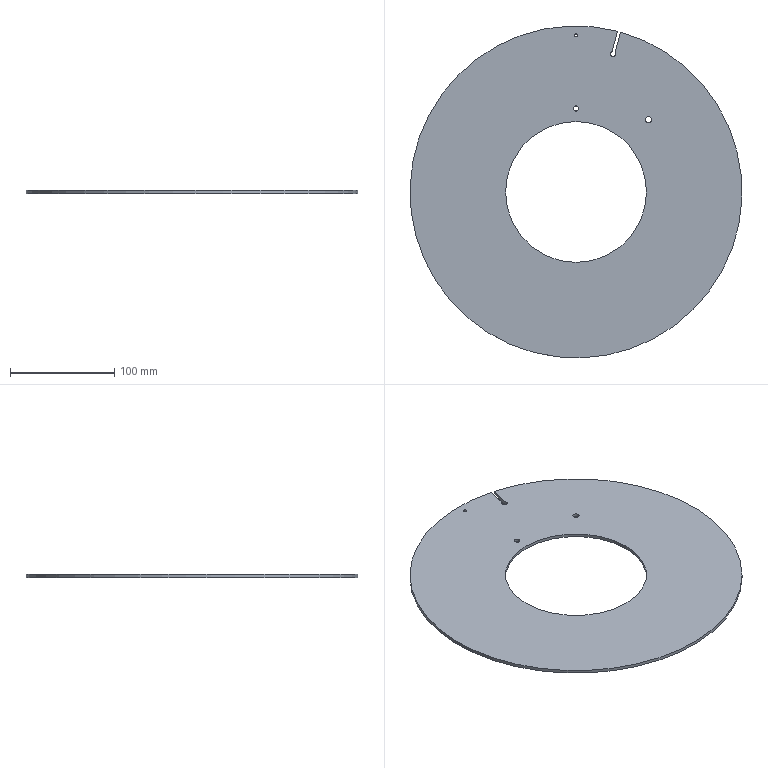Component | NX | SUPPORT_PLATE_1 | 1 solid | 10 faces | box 318 x 318 x 3 mm | volume 194925 mm3 | cylinder 6 | plane 4 | commonest cylinder face diameters 5 x2 318 x1 135 x1 6 x1 3 x1
STEP:
#1=CARTESIAN_POINT('',(0.,0.,0.));
#2=DIRECTION('',(0.,0.,1.));
#3=DIRECTION('',(1.,0.,0.));
#4=AXIS2_PLACEMENT_3D('',#1,#2,#3);
#5=CARTESIAN_POINT('',(42.599,153.187,21.));
#6=VERTEX_POINT('',#5);
#7=CARTESIAN_POINT('',(42.599,153.187,24.));
#8=VERTEX_POINT('',#7);
#9=CARTESIAN_POINT('',(42.599,153.187,20.7));
#10=DIRECTION('',(0.,0.,1.));
#11=VECTOR('',#10,1.);
#12=LINE('',#9,#11);
#13=CARTESIAN_POINT('',(0.,0.,21.));
#14=DIRECTION('',(0.,0.,1.));
#15=DIRECTION('',(1.,0.,0.));
#16=AXIS2_PLACEMENT_3D('',#13,#14,#15);
#17=CYLINDRICAL_SURFACE('',#16,159.);
#18=CARTESIAN_POINT('',(7.583,-0.3));
#19=DIRECTION('',(0.,1.));
#20=VECTOR('',#19,1.);
#21=LINE('',#18,#20);
#22=(GEOMETRIC_REPRESENTATION_CONTEXT(2)PARAMETRIC_REPRESENTATION_CONTEXT()REPRESENTATION_CONTEXT('',''));
#23=DEFINITIONAL_REPRESENTATION('',(#21),#22);
#24=PCURVE('',#17,#23);
#25=CARTESIAN_POINT('',(42.599,153.187,20.7));
#26=DIRECTION('',(-0.9659,0.2588,0.));
#27=DIRECTION('',(0.2588,0.9659,0.));
#28=AXIS2_PLACEMENT_3D('',#25,#26,#27);
#29=PLANE('',#28);
#30=CARTESIAN_POINT('',(0.,0.));
#31=DIRECTION('',(0.,-1.));
#32=VECTOR('',#31,1.);
#33=LINE('',#30,#32);
#34=(GEOMETRIC_REPRESENTATION_CONTEXT(2)PARAMETRIC_REPRESENTATION_CONTEXT()REPRESENTATION_CONTEXT('',''));
#35=DEFINITIONAL_REPRESENTATION('',(#33),#34);
#36=PCURVE('',#29,#35);
#37=SURFACE_CURVE('',#12,(#24,#36),.PCURVE_S1.);
#38=EDGE_CURVE('',#6,#8,#37,.T.);
#39=ORIENTED_EDGE('',*,*,#38,.T.);
#40=CARTESIAN_POINT('',(39.702,153.964,24.));
#41=VERTEX_POINT('',#40);
#42=CARTESIAN_POINT('',(0.,0.,24.));
#43=DIRECTION('',(0.,0.,-1.));
#44=DIRECTION('',(-1.,0.,0.));
#45=AXIS2_PLACEMENT_3D('',#42,#43,#44);
#46=CIRCLE('',#45,159.);
#47=CARTESIAN_POINT('',(9.425,3.));
#48=DIRECTION('',(-1.,0.));
#49=VECTOR('',#48,1.);
#50=LINE('',#47,#49);
#51=(GEOMETRIC_REPRESENTATION_CONTEXT(2)PARAMETRIC_REPRESENTATION_CONTEXT()REPRESENTATION_CONTEXT('',''));
#52=DEFINITIONAL_REPRESENTATION('',(#50),#51);
#53=PCURVE('',#17,#52);
#54=CARTESIAN_POINT('',(0.,0.,24.));
#55=DIRECTION('',(0.,0.,-1.));
#56=DIRECTION('',(-1.,0.,0.));
#57=AXIS2_PLACEMENT_3D('',#54,#55,#56);
#58=PLANE('',#57);
#59=CARTESIAN_POINT('',(0.,0.));
#60=DIRECTION('',(1.,0.));
#61=AXIS2_PLACEMENT_2D('',#59,#60);
#62=CIRCLE('',#61,159.);
#63=(GEOMETRIC_REPRESENTATION_CONTEXT(2)PARAMETRIC_REPRESENTATION_CONTEXT()REPRESENTATION_CONTEXT('',''));
#64=DEFINITIONAL_REPRESENTATION('',(#62),#63);
#65=PCURVE('',#58,#64);
#66=SURFACE_CURVE('',#46,(#53,#65),.PCURVE_S1.);
#67=EDGE_CURVE('',#8,#41,#66,.T.);
#68=ORIENTED_EDGE('',*,*,#67,.T.);
#69=CARTESIAN_POINT('',(39.702,153.964,21.));
#70=VERTEX_POINT('',#69);
#71=CARTESIAN_POINT('',(39.702,153.964,20.7));
#72=DIRECTION('',(0.,0.,1.));
#73=VECTOR('',#72,1.);
#74=LINE('',#71,#73);
#75=CARTESIAN_POINT('',(1.318,-0.3));
#76=DIRECTION('',(0.,1.));
#77=VECTOR('',#76,1.);
#78=LINE('',#75,#77);
#79=(GEOMETRIC_REPRESENTATION_CONTEXT(2)PARAMETRIC_REPRESENTATION_CONTEXT()REPRESENTATION_CONTEXT('',''));
#80=DEFINITIONAL_REPRESENTATION('',(#78),#79);
#81=PCURVE('',#17,#80);
#82=CARTESIAN_POINT('',(34.527,134.652,20.7));
#83=DIRECTION('',(0.9659,-0.2588,0.));
#84=DIRECTION('',(-0.2588,-0.9659,0.));
#85=AXIS2_PLACEMENT_3D('',#82,#83,#84);
#86=PLANE('',#85);
#87=CARTESIAN_POINT('',(-19.993,0.));
#88=DIRECTION('',(0.,-1.));
#89=VECTOR('',#88,1.);
#90=LINE('',#87,#89);
#91=(GEOMETRIC_REPRESENTATION_CONTEXT(2)PARAMETRIC_REPRESENTATION_CONTEXT()REPRESENTATION_CONTEXT('',''));
#92=DEFINITIONAL_REPRESENTATION('',(#90),#91);
#93=PCURVE('',#86,#92);
#94=SURFACE_CURVE('',#74,(#81,#93),.PCURVE_S1.);
#95=EDGE_CURVE('',#70,#41,#94,.T.);
#96=ORIENTED_EDGE('',*,*,#95,.F.);
#97=CARTESIAN_POINT('',(0.,0.,21.));
#98=DIRECTION('',(0.,0.,-1.));
#99=DIRECTION('',(-1.,0.,0.));
#100=AXIS2_PLACEMENT_3D('',#97,#98,#99);
#101=CIRCLE('',#100,159.);
#102=CARTESIAN_POINT('',(9.425,0.));
#103=DIRECTION('',(-1.,0.));
#104=VECTOR('',#103,1.);
#105=LINE('',#102,#104);
#106=(GEOMETRIC_REPRESENTATION_CONTEXT(2)PARAMETRIC_REPRESENTATION_CONTEXT()REPRESENTATION_CONTEXT('',''));
#107=DEFINITIONAL_REPRESENTATION('',(#105),#106);
#108=PCURVE('',#17,#107);
#109=CARTESIAN_POINT('',(0.,0.,21.));
#110=DIRECTION('',(0.,0.,-1.));
#111=DIRECTION('',(-1.,0.,0.));
#112=AXIS2_PLACEMENT_3D('',#109,#110,#111);
#113=PLANE('',#112);
#114=CARTESIAN_POINT('',(0.,0.));
#115=DIRECTION('',(1.,0.));
#116=AXIS2_PLACEMENT_2D('',#114,#115);
#117=CIRCLE('',#116,159.);
#118=(GEOMETRIC_REPRESENTATION_CONTEXT(2)PARAMETRIC_REPRESENTATION_CONTEXT()REPRESENTATION_CONTEXT('',''));
#119=DEFINITIONAL_REPRESENTATION('',(#117),#118);
#120=PCURVE('',#113,#119);
#121=SURFACE_CURVE('',#101,(#108,#120),.PCURVE_S1.);
#122=EDGE_CURVE('',#6,#70,#121,.T.);
#123=ORIENTED_EDGE('',*,*,#122,.F.);
#124=EDGE_LOOP('',(#39,#68,#96,#123));
#125=FACE_BOUND('',#124,.T.);
#126=ADVANCED_FACE('',(#125),#17,.T.);
#127=CARTESIAN_POINT('',(-67.5,0.,21.));
#128=VERTEX_POINT('',#127);
#129=CARTESIAN_POINT('',(0.,0.,21.));
#130=DIRECTION('',(0.,0.,-1.));
#131=DIRECTION('',(-1.,0.,0.));
#132=AXIS2_PLACEMENT_3D('',#129,#130,#131);
#133=CIRCLE('',#132,67.5);
#134=CARTESIAN_POINT('',(0.,0.));
#135=DIRECTION('',(1.,0.));
#136=AXIS2_PLACEMENT_2D('',#134,#135);
#137=CIRCLE('',#136,67.5);
#138=(GEOMETRIC_REPRESENTATION_CONTEXT(2)PARAMETRIC_REPRESENTATION_CONTEXT()REPRESENTATION_CONTEXT('',''));
#139=DEFINITIONAL_REPRESENTATION('',(#137),#138);
#140=PCURVE('',#113,#139);
#141=CARTESIAN_POINT('',(0.,0.,21.));
#142=DIRECTION('',(0.,0.,1.));
#143=DIRECTION('',(1.,0.,0.));
#144=AXIS2_PLACEMENT_3D('',#141,#142,#143);
#145=CYLINDRICAL_SURFACE('',#144,67.5);
#146=CARTESIAN_POINT('',(9.425,0.));
#147=DIRECTION('',(-1.,0.));
#148=VECTOR('',#147,1.);
#149=LINE('',#146,#148);
#150=(GEOMETRIC_REPRESENTATION_CONTEXT(2)PARAMETRIC_REPRESENTATION_CONTEXT()REPRESENTATION_CONTEXT('',''));
#151=DEFINITIONAL_REPRESENTATION('',(#149),#150);
#152=PCURVE('',#145,#151);
#153=SURFACE_CURVE('',#133,(#140,#152),.PCURVE_S1.);
#154=EDGE_CURVE('',#128,#128,#153,.T.);
#155=ORIENTED_EDGE('',*,*,#154,.F.);
#156=EDGE_LOOP('',(#155));
#157=FACE_BOUND('',#156,.T.);
#158=CARTESIAN_POINT('',(2.5,80.,21.));
#159=VERTEX_POINT('',#158);
#160=CARTESIAN_POINT('',(0.,80.,21.));
#161=DIRECTION('',(0.,0.,1.));
#162=DIRECTION('',(1.,0.,0.));
#163=AXIS2_PLACEMENT_3D('',#160,#161,#162);
#164=CIRCLE('',#163,2.5);
#165=CARTESIAN_POINT('',(-2.5,80.));
#166=CARTESIAN_POINT('',(-2.5,84.33));
#167=CARTESIAN_POINT('',(1.25,82.165));
#168=CARTESIAN_POINT('',(5.,80.));
#169=CARTESIAN_POINT('',(1.25,77.835));
#170=CARTESIAN_POINT('',(-2.5,75.67));
#171=CARTESIAN_POINT('',(-2.5,80.));
#172=(BOUNDED_CURVE()B_SPLINE_CURVE(2,(#165,#166,#167,#168,#169,#170,#171),.UNSPECIFIED.,.T.,.F.)B_SPLINE_CURVE_WITH_KNOTS((1,2,2,2,2,1),(-2.094,0.,2.094,4.189,6.283,8.378),.UNSPECIFIED.)CURVE()GEOMETRIC_REPRESENTATION_ITEM()RATIONAL_B_SPLINE_CURVE((1.,0.5,1.,0.5,1.,0.5,1.))REPRESENTATION_ITEM(''));
#173=(GEOMETRIC_REPRESENTATION_CONTEXT(2)PARAMETRIC_REPRESENTATION_CONTEXT()REPRESENTATION_CONTEXT('',''));
#174=DEFINITIONAL_REPRESENTATION('',(#172),#173);
#175=PCURVE('',#113,#174);
#176=CARTESIAN_POINT('',(0.,80.,21.));
#177=DIRECTION('',(0.,0.,1.));
#178=DIRECTION('',(1.,0.,0.));
#179=AXIS2_PLACEMENT_3D('',#176,#177,#178);
#180=CYLINDRICAL_SURFACE('',#179,2.5);
#181=CARTESIAN_POINT('',(0.,0.));
#182=DIRECTION('',(1.,0.));
#183=VECTOR('',#182,1.);
#184=LINE('',#181,#183);
#185=(GEOMETRIC_REPRESENTATION_CONTEXT(2)PARAMETRIC_REPRESENTATION_CONTEXT()REPRESENTATION_CONTEXT('',''));
#186=DEFINITIONAL_REPRESENTATION('',(#184),#185);
#187=PCURVE('',#180,#186);
#188=SURFACE_CURVE('',#164,(#175,#187),.PCURVE_S1.);
#189=EDGE_CURVE('',#159,#159,#188,.T.);
#190=ORIENTED_EDGE('',*,*,#189,.T.);
#191=EDGE_LOOP('',(#190));
#192=FACE_BOUND('',#191,.T.);
#193=CARTESIAN_POINT('',(72.296,69.296,21.));
#194=VERTEX_POINT('',#193);
#195=CARTESIAN_POINT('',(69.296,69.296,21.));
#196=DIRECTION('',(0.,0.,1.));
#197=DIRECTION('',(1.,0.,0.));
#198=AXIS2_PLACEMENT_3D('',#195,#196,#197);
#199=CIRCLE('',#198,3.);
#200=CARTESIAN_POINT('',(-72.296,69.296));
#201=CARTESIAN_POINT('',(-72.296,74.493));
#202=CARTESIAN_POINT('',(-67.796,71.895));
#203=CARTESIAN_POINT('',(-63.296,69.296));
#204=CARTESIAN_POINT('',(-67.796,66.698));
#205=CARTESIAN_POINT('',(-72.296,64.1));
#206=CARTESIAN_POINT('',(-72.296,69.296));
#207=(BOUNDED_CURVE()B_SPLINE_CURVE(2,(#200,#201,#202,#203,#204,#205,#206),.UNSPECIFIED.,.T.,.F.)B_SPLINE_CURVE_WITH_KNOTS((1,2,2,2,2,1),(-2.094,0.,2.094,4.189,6.283,8.378),.UNSPECIFIED.)CURVE()GEOMETRIC_REPRESENTATION_ITEM()RATIONAL_B_SPLINE_CURVE((1.,0.5,1.,0.5,1.,0.5,1.))REPRESENTATION_ITEM(''));
#208=(GEOMETRIC_REPRESENTATION_CONTEXT(2)PARAMETRIC_REPRESENTATION_CONTEXT()REPRESENTATION_CONTEXT('',''));
#209=DEFINITIONAL_REPRESENTATION('',(#207),#208);
#210=PCURVE('',#113,#209);
#211=CARTESIAN_POINT('',(69.296,69.296,21.));
#212=DIRECTION('',(0.,0.,1.));
#213=DIRECTION('',(1.,0.,0.));
#214=AXIS2_PLACEMENT_3D('',#211,#212,#213);
#215=CYLINDRICAL_SURFACE('',#214,3.);
#216=CARTESIAN_POINT('',(0.,0.));
#217=DIRECTION('',(1.,0.));
#218=VECTOR('',#217,1.);
#219=LINE('',#216,#218);
#220=(GEOMETRIC_REPRESENTATION_CONTEXT(2)PARAMETRIC_REPRESENTATION_CONTEXT()REPRESENTATION_CONTEXT('',''));
#221=DEFINITIONAL_REPRESENTATION('',(#219),#220);
#222=PCURVE('',#215,#221);
#223=SURFACE_CURVE('',#199,(#210,#222),.PCURVE_S1.);
#224=EDGE_CURVE('',#194,#194,#223,.T.);
#225=ORIENTED_EDGE('',*,*,#224,.T.);
#226=EDGE_LOOP('',(#225));
#227=FACE_BOUND('',#226,.T.);
#228=CARTESIAN_POINT('',(1.5,150.,21.));
#229=VERTEX_POINT('',#228);
#230=CARTESIAN_POINT('',(0.,150.,21.));
#231=DIRECTION('',(0.,0.,1.));
#232=DIRECTION('',(1.,0.,0.));
#233=AXIS2_PLACEMENT_3D('',#230,#231,#232);
#234=CIRCLE('',#233,1.5);
#235=CARTESIAN_POINT('',(-1.5,150.));
#236=CARTESIAN_POINT('',(-1.5,152.598));
#237=CARTESIAN_POINT('',(0.75,151.299));
#238=CARTESIAN_POINT('',(3.,150.));
#239=CARTESIAN_POINT('',(0.75,148.701));
#240=CARTESIAN_POINT('',(-1.5,147.402));
#241=CARTESIAN_POINT('',(-1.5,150.));
#242=(BOUNDED_CURVE()B_SPLINE_CURVE(2,(#235,#236,#237,#238,#239,#240,#241),.UNSPECIFIED.,.T.,.F.)B_SPLINE_CURVE_WITH_KNOTS((1,2,2,2,2,1),(-2.094,0.,2.094,4.189,6.283,8.378),.UNSPECIFIED.)CURVE()GEOMETRIC_REPRESENTATION_ITEM()RATIONAL_B_SPLINE_CURVE((1.,0.5,1.,0.5,1.,0.5,1.))REPRESENTATION_ITEM(''));
#243=(GEOMETRIC_REPRESENTATION_CONTEXT(2)PARAMETRIC_REPRESENTATION_CONTEXT()REPRESENTATION_CONTEXT('',''));
#244=DEFINITIONAL_REPRESENTATION('',(#242),#243);
#245=PCURVE('',#113,#244);
#246=CARTESIAN_POINT('',(0.,150.,21.));
#247=DIRECTION('',(0.,0.,1.));
#248=DIRECTION('',(1.,0.,0.));
#249=AXIS2_PLACEMENT_3D('',#246,#247,#248);
#250=CYLINDRICAL_SURFACE('',#249,1.5);
#251=CARTESIAN_POINT('',(0.,0.));
#252=DIRECTION('',(1.,0.));
#253=VECTOR('',#252,1.);
#254=LINE('',#251,#253);
#255=(GEOMETRIC_REPRESENTATION_CONTEXT(2)PARAMETRIC_REPRESENTATION_CONTEXT()REPRESENTATION_CONTEXT('',''));
#256=DEFINITIONAL_REPRESENTATION('',(#254),#255);
#257=PCURVE('',#250,#256);
#258=SURFACE_CURVE('',#234,(#245,#257),.PCURVE_S1.);
#259=EDGE_CURVE('',#229,#229,#258,.T.);
#260=ORIENTED_EDGE('',*,*,#259,.T.);
#261=EDGE_LOOP('',(#260));
#262=FACE_BOUND('',#261,.T.);
#263=CARTESIAN_POINT('',(34.527,134.652,21.));
#264=VERTEX_POINT('',#263);
#265=CARTESIAN_POINT('',(37.425,133.875,21.));
#266=VERTEX_POINT('',#265);
#267=CARTESIAN_POINT('',(35.458,132.332,21.));
#268=DIRECTION('',(0.,0.,1.));
#269=DIRECTION('',(-1.,0.,0.));
#270=AXIS2_PLACEMENT_3D('',#267,#268,#269);
#271=CIRCLE('',#270,2.5);
#272=CARTESIAN_POINT('',(-32.958,132.332));
#273=CARTESIAN_POINT('',(-32.958,128.002));
#274=CARTESIAN_POINT('',(-36.708,130.167));
#275=CARTESIAN_POINT('',(-40.458,132.332));
#276=CARTESIAN_POINT('',(-36.708,134.497));
#277=CARTESIAN_POINT('',(-32.958,136.662));
#278=CARTESIAN_POINT('',(-32.958,132.332));
#279=(BOUNDED_CURVE()B_SPLINE_CURVE(2,(#272,#273,#274,#275,#276,#277,#278),.UNSPECIFIED.,.T.,.F.)B_SPLINE_CURVE_WITH_KNOTS((1,2,2,2,2,1),(-2.094,0.,2.094,4.189,6.283,8.378),.UNSPECIFIED.)CURVE()GEOMETRIC_REPRESENTATION_ITEM()RATIONAL_B_SPLINE_CURVE((1.,0.5,1.,0.5,1.,0.5,1.))REPRESENTATION_ITEM(''));
#280=(GEOMETRIC_REPRESENTATION_CONTEXT(2)PARAMETRIC_REPRESENTATION_CONTEXT()REPRESENTATION_CONTEXT('',''));
#281=DEFINITIONAL_REPRESENTATION('',(#279),#280);
#282=PCURVE('',#113,#281);
#283=CARTESIAN_POINT('',(35.458,132.332,20.7));
#284=DIRECTION('',(0.,0.,1.));
#285=DIRECTION('',(1.,0.,0.));
#286=AXIS2_PLACEMENT_3D('',#283,#284,#285);
#287=CYLINDRICAL_SURFACE('',#286,2.5);
#288=CARTESIAN_POINT('',(-3.142,0.3));
#289=DIRECTION('',(1.,0.));
#290=VECTOR('',#289,1.);
#291=LINE('',#288,#290);
#292=(GEOMETRIC_REPRESENTATION_CONTEXT(2)PARAMETRIC_REPRESENTATION_CONTEXT()REPRESENTATION_CONTEXT('',''));
#293=DEFINITIONAL_REPRESENTATION('',(#291),#292);
#294=PCURVE('',#287,#293);
#295=SURFACE_CURVE('',#271,(#282,#294),.PCURVE_S1.);
#296=EDGE_CURVE('',#264,#266,#295,.T.);
#297=ORIENTED_EDGE('',*,*,#296,.T.);
#298=CARTESIAN_POINT('',(1.449,-0.3882,21.));
#299=DIRECTION('',(0.2588,0.9659,0.));
#300=VECTOR('',#299,1.);
#301=LINE('',#298,#300);
#302=CARTESIAN_POINT('',(-1.449,-0.3882));
#303=DIRECTION('',(-0.2588,0.9659));
#304=VECTOR('',#303,1.);
#305=LINE('',#302,#304);
#306=(GEOMETRIC_REPRESENTATION_CONTEXT(2)PARAMETRIC_REPRESENTATION_CONTEXT()REPRESENTATION_CONTEXT('',''));
#307=DEFINITIONAL_REPRESENTATION('',(#305),#306);
#308=PCURVE('',#113,#307);
#309=CARTESIAN_POINT('',(-158.993,-0.3));
#310=DIRECTION('',(1.,0.));
#311=VECTOR('',#310,1.);
#312=LINE('',#309,#311);
#313=(GEOMETRIC_REPRESENTATION_CONTEXT(2)PARAMETRIC_REPRESENTATION_CONTEXT()REPRESENTATION_CONTEXT('',''));
#314=DEFINITIONAL_REPRESENTATION('',(#312),#313);
#315=PCURVE('',#29,#314);
#316=SURFACE_CURVE('',#301,(#308,#315),.PCURVE_S1.);
#317=EDGE_CURVE('',#266,#6,#316,.T.);
#318=ORIENTED_EDGE('',*,*,#317,.T.);
#319=ORIENTED_EDGE('',*,*,#122,.T.);
#320=CARTESIAN_POINT('',(-1.449,0.3882,21.));
#321=DIRECTION('',(-0.2588,-0.9659,0.));
#322=VECTOR('',#321,1.);
#323=LINE('',#320,#322);
#324=CARTESIAN_POINT('',(1.449,0.3882));
#325=DIRECTION('',(0.2588,-0.9659));
#326=VECTOR('',#325,1.);
#327=LINE('',#324,#326);
#328=(GEOMETRIC_REPRESENTATION_CONTEXT(2)PARAMETRIC_REPRESENTATION_CONTEXT()REPRESENTATION_CONTEXT('',''));
#329=DEFINITIONAL_REPRESENTATION('',(#327),#328);
#330=PCURVE('',#113,#329);
#331=CARTESIAN_POINT('',(139.,-0.3));
#332=DIRECTION('',(1.,0.));
#333=VECTOR('',#332,1.);
#334=LINE('',#331,#333);
#335=(GEOMETRIC_REPRESENTATION_CONTEXT(2)PARAMETRIC_REPRESENTATION_CONTEXT()REPRESENTATION_CONTEXT('',''));
#336=DEFINITIONAL_REPRESENTATION('',(#334),#335);
#337=PCURVE('',#86,#336);
#338=SURFACE_CURVE('',#323,(#330,#337),.PCURVE_S1.);
#339=EDGE_CURVE('',#70,#264,#338,.T.);
#340=ORIENTED_EDGE('',*,*,#339,.T.);
#341=EDGE_LOOP('',(#297,#318,#319,#340));
#342=FACE_BOUND('',#341,.T.);
#343=ADVANCED_FACE('',(#157,#192,#227,#262,#342),#113,.T.);
#344=ORIENTED_EDGE('',*,*,#154,.F.);
#345=CARTESIAN_POINT('',(-67.5,0.,24.));
#346=VERTEX_POINT('',#345);
#347=CARTESIAN_POINT('',(-67.5,0.,21.));
#348=CARTESIAN_POINT('',(-67.5,0.,24.));
#349=B_SPLINE_CURVE_WITH_KNOTS('',1,(#347,#348),.UNSPECIFIED.,.F.,.F.,(2,2),(0.,3.),.PIECEWISE_BEZIER_KNOTS.);
#350=CARTESIAN_POINT('',(9.425,0.));
#351=DIRECTION('',(0.,1.));
#352=VECTOR('',#351,1.);
#353=LINE('',#350,#352);
#354=(GEOMETRIC_REPRESENTATION_CONTEXT(2)PARAMETRIC_REPRESENTATION_CONTEXT()REPRESENTATION_CONTEXT('',''));
#355=DEFINITIONAL_REPRESENTATION('',(#353),#354);
#356=PCURVE('',#145,#355);
#357=CARTESIAN_POINT('',(3.142,0.));
#358=DIRECTION('',(0.,1.));
#359=VECTOR('',#358,1.);
#360=LINE('',#357,#359);
#361=(GEOMETRIC_REPRESENTATION_CONTEXT(2)PARAMETRIC_REPRESENTATION_CONTEXT()REPRESENTATION_CONTEXT('',''));
#362=DEFINITIONAL_REPRESENTATION('',(#360),#361);
#363=PCURVE('',#145,#362);
#364=SEAM_CURVE('',#349,(#356,#363),.PCURVE_S1.);
#365=EDGE_CURVE('',#128,#346,#364,.T.);
#366=ORIENTED_EDGE('',*,*,#365,.T.);
#367=CARTESIAN_POINT('',(0.,0.,24.));
#368=DIRECTION('',(0.,0.,-1.));
#369=DIRECTION('',(-1.,0.,0.));
#370=AXIS2_PLACEMENT_3D('',#367,#368,#369);
#371=CIRCLE('',#370,67.5);
#372=CARTESIAN_POINT('',(9.425,3.));
#373=DIRECTION('',(-1.,0.));
#374=VECTOR('',#373,1.);
#375=LINE('',#372,#374);
#376=(GEOMETRIC_REPRESENTATION_CONTEXT(2)PARAMETRIC_REPRESENTATION_CONTEXT()REPRESENTATION_CONTEXT('',''));
#377=DEFINITIONAL_REPRESENTATION('',(#375),#376);
#378=PCURVE('',#145,#377);
#379=CARTESIAN_POINT('',(0.,0.));
#380=DIRECTION('',(1.,0.));
#381=AXIS2_PLACEMENT_2D('',#379,#380);
#382=CIRCLE('',#381,67.5);
#383=(GEOMETRIC_REPRESENTATION_CONTEXT(2)PARAMETRIC_REPRESENTATION_CONTEXT()REPRESENTATION_CONTEXT('',''));
#384=DEFINITIONAL_REPRESENTATION('',(#382),#383);
#385=PCURVE('',#58,#384);
#386=SURFACE_CURVE('',#371,(#378,#385),.PCURVE_S1.);
#387=EDGE_CURVE('',#346,#346,#386,.T.);
#388=ORIENTED_EDGE('',*,*,#387,.T.);
#389=ORIENTED_EDGE('',*,*,#365,.F.);
#390=EDGE_LOOP('',(#344,#366,#388,#389));
#391=FACE_BOUND('',#390,.F.);
#392=ADVANCED_FACE('',(#391),#145,.F.);
#393=CARTESIAN_POINT('',(1.5,150.,24.));
#394=VERTEX_POINT('',#393);
#395=CARTESIAN_POINT('',(0.,150.,24.));
#396=DIRECTION('',(0.,0.,1.));
#397=DIRECTION('',(1.,0.,0.));
#398=AXIS2_PLACEMENT_3D('',#395,#396,#397);
#399=CIRCLE('',#398,1.5);
#400=CARTESIAN_POINT('',(-1.5,150.));
#401=CARTESIAN_POINT('',(-1.5,152.598));
#402=CARTESIAN_POINT('',(0.75,151.299));
#403=CARTESIAN_POINT('',(3.,150.));
#404=CARTESIAN_POINT('',(0.75,148.701));
#405=CARTESIAN_POINT('',(-1.5,147.402));
#406=CARTESIAN_POINT('',(-1.5,150.));
#407=(BOUNDED_CURVE()B_SPLINE_CURVE(2,(#400,#401,#402,#403,#404,#405,#406),.UNSPECIFIED.,.T.,.F.)B_SPLINE_CURVE_WITH_KNOTS((1,2,2,2,2,1),(-2.094,0.,2.094,4.189,6.283,8.378),.UNSPECIFIED.)CURVE()GEOMETRIC_REPRESENTATION_ITEM()RATIONAL_B_SPLINE_CURVE((1.,0.5,1.,0.5,1.,0.5,1.))REPRESENTATION_ITEM(''));
#408=(GEOMETRIC_REPRESENTATION_CONTEXT(2)PARAMETRIC_REPRESENTATION_CONTEXT()REPRESENTATION_CONTEXT('',''));
#409=DEFINITIONAL_REPRESENTATION('',(#407),#408);
#410=PCURVE('',#58,#409);
#411=CARTESIAN_POINT('',(0.,3.));
#412=DIRECTION('',(1.,0.));
#413=VECTOR('',#412,1.);
#414=LINE('',#411,#413);
#415=(GEOMETRIC_REPRESENTATION_CONTEXT(2)PARAMETRIC_REPRESENTATION_CONTEXT()REPRESENTATION_CONTEXT('',''));
#416=DEFINITIONAL_REPRESENTATION('',(#414),#415);
#417=PCURVE('',#250,#416);
#418=SURFACE_CURVE('',#399,(#410,#417),.PCURVE_S1.);
#419=EDGE_CURVE('',#394,#394,#418,.T.);
#420=ORIENTED_EDGE('',*,*,#419,.F.);
#421=EDGE_LOOP('',(#420));
#422=FACE_BOUND('',#421,.T.);
#423=CARTESIAN_POINT('',(72.296,69.296,24.));
#424=VERTEX_POINT('',#423);
#425=CARTESIAN_POINT('',(69.296,69.296,24.));
#426=DIRECTION('',(0.,0.,1.));
#427=DIRECTION('',(1.,0.,0.));
#428=AXIS2_PLACEMENT_3D('',#425,#426,#427);
#429=CIRCLE('',#428,3.);
#430=CARTESIAN_POINT('',(-72.296,69.296));
#431=CARTESIAN_POINT('',(-72.296,74.493));
#432=CARTESIAN_POINT('',(-67.796,71.895));
#433=CARTESIAN_POINT('',(-63.296,69.296));
#434=CARTESIAN_POINT('',(-67.796,66.698));
#435=CARTESIAN_POINT('',(-72.296,64.1));
#436=CARTESIAN_POINT('',(-72.296,69.296));
#437=(BOUNDED_CURVE()B_SPLINE_CURVE(2,(#430,#431,#432,#433,#434,#435,#436),.UNSPECIFIED.,.T.,.F.)B_SPLINE_CURVE_WITH_KNOTS((1,2,2,2,2,1),(-2.094,0.,2.094,4.189,6.283,8.378),.UNSPECIFIED.)CURVE()GEOMETRIC_REPRESENTATION_ITEM()RATIONAL_B_SPLINE_CURVE((1.,0.5,1.,0.5,1.,0.5,1.))REPRESENTATION_ITEM(''));
#438=(GEOMETRIC_REPRESENTATION_CONTEXT(2)PARAMETRIC_REPRESENTATION_CONTEXT()REPRESENTATION_CONTEXT('',''));
#439=DEFINITIONAL_REPRESENTATION('',(#437),#438);
#440=PCURVE('',#58,#439);
#441=CARTESIAN_POINT('',(0.,3.));
#442=DIRECTION('',(1.,0.));
#443=VECTOR('',#442,1.);
#444=LINE('',#441,#443);
#445=(GEOMETRIC_REPRESENTATION_CONTEXT(2)PARAMETRIC_REPRESENTATION_CONTEXT()REPRESENTATION_CONTEXT('',''));
#446=DEFINITIONAL_REPRESENTATION('',(#444),#445);
#447=PCURVE('',#215,#446);
#448=SURFACE_CURVE('',#429,(#440,#447),.PCURVE_S1.);
#449=EDGE_CURVE('',#424,#424,#448,.T.);
#450=ORIENTED_EDGE('',*,*,#449,.F.);
#451=EDGE_LOOP('',(#450));
#452=FACE_BOUND('',#451,.T.);
#453=CARTESIAN_POINT('',(2.5,80.,24.));
#454=VERTEX_POINT('',#453);
#455=CARTESIAN_POINT('',(0.,80.,24.));
#456=DIRECTION('',(0.,0.,1.));
#457=DIRECTION('',(1.,0.,0.));
#458=AXIS2_PLACEMENT_3D('',#455,#456,#457);
#459=CIRCLE('',#458,2.5);
#460=CARTESIAN_POINT('',(-2.5,80.));
#461=CARTESIAN_POINT('',(-2.5,84.33));
#462=CARTESIAN_POINT('',(1.25,82.165));
#463=CARTESIAN_POINT('',(5.,80.));
#464=CARTESIAN_POINT('',(1.25,77.835));
#465=CARTESIAN_POINT('',(-2.5,75.67));
#466=CARTESIAN_POINT('',(-2.5,80.));
#467=(BOUNDED_CURVE()B_SPLINE_CURVE(2,(#460,#461,#462,#463,#464,#465,#466),.UNSPECIFIED.,.T.,.F.)B_SPLINE_CURVE_WITH_KNOTS((1,2,2,2,2,1),(-2.094,0.,2.094,4.189,6.283,8.378),.UNSPECIFIED.)CURVE()GEOMETRIC_REPRESENTATION_ITEM()RATIONAL_B_SPLINE_CURVE((1.,0.5,1.,0.5,1.,0.5,1.))REPRESENTATION_ITEM(''));
#468=(GEOMETRIC_REPRESENTATION_CONTEXT(2)PARAMETRIC_REPRESENTATION_CONTEXT()REPRESENTATION_CONTEXT('',''));
#469=DEFINITIONAL_REPRESENTATION('',(#467),#468);
#470=PCURVE('',#58,#469);
#471=CARTESIAN_POINT('',(0.,3.));
#472=DIRECTION('',(1.,0.));
#473=VECTOR('',#472,1.);
#474=LINE('',#471,#473);
#475=(GEOMETRIC_REPRESENTATION_CONTEXT(2)PARAMETRIC_REPRESENTATION_CONTEXT()REPRESENTATION_CONTEXT('',''));
#476=DEFINITIONAL_REPRESENTATION('',(#474),#475);
#477=PCURVE('',#180,#476);
#478=SURFACE_CURVE('',#459,(#470,#477),.PCURVE_S1.);
#479=EDGE_CURVE('',#454,#454,#478,.T.);
#480=ORIENTED_EDGE('',*,*,#479,.F.);
#481=EDGE_LOOP('',(#480));
#482=FACE_BOUND('',#481,.T.);
#483=CARTESIAN_POINT('',(37.425,133.875,24.));
#484=VERTEX_POINT('',#483);
#485=CARTESIAN_POINT('',(34.527,134.652,24.));
#486=VERTEX_POINT('',#485);
#487=CARTESIAN_POINT('',(35.458,132.332,24.));
#488=DIRECTION('',(0.,0.,-1.));
#489=DIRECTION('',(-1.,0.,0.));
#490=AXIS2_PLACEMENT_3D('',#487,#488,#489);
#491=CIRCLE('',#490,2.5);
#492=CARTESIAN_POINT('',(-35.458,132.332));
#493=DIRECTION('',(1.,0.));
#494=AXIS2_PLACEMENT_2D('',#492,#493);
#495=CIRCLE('',#494,2.5);
#496=(GEOMETRIC_REPRESENTATION_CONTEXT(2)PARAMETRIC_REPRESENTATION_CONTEXT()REPRESENTATION_CONTEXT('',''));
#497=DEFINITIONAL_REPRESENTATION('',(#495),#496);
#498=PCURVE('',#58,#497);
#499=CARTESIAN_POINT('',(9.425,3.3));
#500=DIRECTION('',(-1.,0.));
#501=VECTOR('',#500,1.);
#502=LINE('',#499,#501);
#503=(GEOMETRIC_REPRESENTATION_CONTEXT(2)PARAMETRIC_REPRESENTATION_CONTEXT()REPRESENTATION_CONTEXT('',''));
#504=DEFINITIONAL_REPRESENTATION('',(#502),#503);
#505=PCURVE('',#287,#504);
#506=SURFACE_CURVE('',#491,(#498,#505),.PCURVE_S1.);
#507=EDGE_CURVE('',#484,#486,#506,.T.);
#508=ORIENTED_EDGE('',*,*,#507,.T.);
#509=CARTESIAN_POINT('',(34.527,134.652,24.));
#510=DIRECTION('',(0.2588,0.9659,0.));
#511=VECTOR('',#510,1.);
#512=LINE('',#509,#511);
#513=CARTESIAN_POINT('',(-34.527,134.652));
#514=DIRECTION('',(-0.2588,0.9659));
#515=VECTOR('',#514,1.);
#516=LINE('',#513,#515);
#517=(GEOMETRIC_REPRESENTATION_CONTEXT(2)PARAMETRIC_REPRESENTATION_CONTEXT()REPRESENTATION_CONTEXT('',''));
#518=DEFINITIONAL_REPRESENTATION('',(#516),#517);
#519=PCURVE('',#58,#518);
#520=CARTESIAN_POINT('',(0.,-3.3));
#521=DIRECTION('',(-1.,0.));
#522=VECTOR('',#521,1.);
#523=LINE('',#520,#522);
#524=(GEOMETRIC_REPRESENTATION_CONTEXT(2)PARAMETRIC_REPRESENTATION_CONTEXT()REPRESENTATION_CONTEXT('',''));
#525=DEFINITIONAL_REPRESENTATION('',(#523),#524);
#526=PCURVE('',#86,#525);
#527=SURFACE_CURVE('',#512,(#519,#526),.PCURVE_S1.);
#528=EDGE_CURVE('',#486,#41,#527,.T.);
#529=ORIENTED_EDGE('',*,*,#528,.T.);
#530=ORIENTED_EDGE('',*,*,#67,.F.);
#531=CARTESIAN_POINT('',(42.599,153.187,24.));
#532=DIRECTION('',(-0.2588,-0.9659,0.));
#533=VECTOR('',#532,1.);
#534=LINE('',#531,#533);
#535=CARTESIAN_POINT('',(-42.599,153.187));
#536=DIRECTION('',(0.2588,-0.9659));
#537=VECTOR('',#536,1.);
#538=LINE('',#535,#537);
#539=(GEOMETRIC_REPRESENTATION_CONTEXT(2)PARAMETRIC_REPRESENTATION_CONTEXT()REPRESENTATION_CONTEXT('',''));
#540=DEFINITIONAL_REPRESENTATION('',(#538),#539);
#541=PCURVE('',#58,#540);
#542=CARTESIAN_POINT('',(0.,-3.3));
#543=DIRECTION('',(-1.,0.));
#544=VECTOR('',#543,1.);
#545=LINE('',#542,#544);
#546=(GEOMETRIC_REPRESENTATION_CONTEXT(2)PARAMETRIC_REPRESENTATION_CONTEXT()REPRESENTATION_CONTEXT('',''));
#547=DEFINITIONAL_REPRESENTATION('',(#545),#546);
#548=PCURVE('',#29,#547);
#549=SURFACE_CURVE('',#534,(#541,#548),.PCURVE_S1.);
#550=EDGE_CURVE('',#8,#484,#549,.T.);
#551=ORIENTED_EDGE('',*,*,#550,.T.);
#552=EDGE_LOOP('',(#508,#529,#530,#551));
#553=FACE_BOUND('',#552,.T.);
#554=ORIENTED_EDGE('',*,*,#387,.T.);
#555=EDGE_LOOP('',(#554));
#556=FACE_BOUND('',#555,.T.);
#557=ADVANCED_FACE('',(#422,#452,#482,#553,#556),#58,.F.);
#558=ORIENTED_EDGE('',*,*,#479,.F.);
#559=CARTESIAN_POINT('',(2.5,80.,21.));
#560=CARTESIAN_POINT('',(2.5,80.,24.));
#561=B_SPLINE_CURVE_WITH_KNOTS('',1,(#559,#560),.UNSPECIFIED.,.F.,.F.,(2,2),(0.,3.),.PIECEWISE_BEZIER_KNOTS.);
#562=CARTESIAN_POINT('',(0.,0.));
#563=DIRECTION('',(0.,1.));
#564=VECTOR('',#563,1.);
#565=LINE('',#562,#564);
#566=(GEOMETRIC_REPRESENTATION_CONTEXT(2)PARAMETRIC_REPRESENTATION_CONTEXT()REPRESENTATION_CONTEXT('',''));
#567=DEFINITIONAL_REPRESENTATION('',(#565),#566);
#568=PCURVE('',#180,#567);
#569=CARTESIAN_POINT('',(6.283,0.));
#570=DIRECTION('',(0.,1.));
#571=VECTOR('',#570,1.);
#572=LINE('',#569,#571);
#573=(GEOMETRIC_REPRESENTATION_CONTEXT(2)PARAMETRIC_REPRESENTATION_CONTEXT()REPRESENTATION_CONTEXT('',''));
#574=DEFINITIONAL_REPRESENTATION('',(#572),#573);
#575=PCURVE('',#180,#574);
#576=SEAM_CURVE('',#561,(#568,#575),.PCURVE_S1.);
#577=EDGE_CURVE('',#159,#454,#576,.T.);
#578=ORIENTED_EDGE('',*,*,#577,.F.);
#579=ORIENTED_EDGE('',*,*,#189,.T.);
#580=ORIENTED_EDGE('',*,*,#577,.T.);
#581=EDGE_LOOP('',(#558,#578,#579,#580));
#582=FACE_BOUND('',#581,.F.);
#583=ADVANCED_FACE('',(#582),#180,.F.);
#584=ORIENTED_EDGE('',*,*,#449,.F.);
#585=CARTESIAN_POINT('',(72.296,69.296,21.));
#586=CARTESIAN_POINT('',(72.296,69.296,24.));
#587=B_SPLINE_CURVE_WITH_KNOTS('',1,(#585,#586),.UNSPECIFIED.,.F.,.F.,(2,2),(0.,3.),.PIECEWISE_BEZIER_KNOTS.);
#588=CARTESIAN_POINT('',(0.,0.));
#589=DIRECTION('',(0.,1.));
#590=VECTOR('',#589,1.);
#591=LINE('',#588,#590);
#592=(GEOMETRIC_REPRESENTATION_CONTEXT(2)PARAMETRIC_REPRESENTATION_CONTEXT()REPRESENTATION_CONTEXT('',''));
#593=DEFINITIONAL_REPRESENTATION('',(#591),#592);
#594=PCURVE('',#215,#593);
#595=CARTESIAN_POINT('',(6.283,0.));
#596=DIRECTION('',(0.,1.));
#597=VECTOR('',#596,1.);
#598=LINE('',#595,#597);
#599=(GEOMETRIC_REPRESENTATION_CONTEXT(2)PARAMETRIC_REPRESENTATION_CONTEXT()REPRESENTATION_CONTEXT('',''));
#600=DEFINITIONAL_REPRESENTATION('',(#598),#599);
#601=PCURVE('',#215,#600);
#602=SEAM_CURVE('',#587,(#594,#601),.PCURVE_S1.);
#603=EDGE_CURVE('',#194,#424,#602,.T.);
#604=ORIENTED_EDGE('',*,*,#603,.F.);
#605=ORIENTED_EDGE('',*,*,#224,.T.);
#606=ORIENTED_EDGE('',*,*,#603,.T.);
#607=EDGE_LOOP('',(#584,#604,#605,#606));
#608=FACE_BOUND('',#607,.F.);
#609=ADVANCED_FACE('',(#608),#215,.F.);
#610=ORIENTED_EDGE('',*,*,#419,.F.);
#611=CARTESIAN_POINT('',(1.5,150.,21.));
#612=CARTESIAN_POINT('',(1.5,150.,24.));
#613=B_SPLINE_CURVE_WITH_KNOTS('',1,(#611,#612),.UNSPECIFIED.,.F.,.F.,(2,2),(0.,3.),.PIECEWISE_BEZIER_KNOTS.);
#614=CARTESIAN_POINT('',(0.,0.));
#615=DIRECTION('',(0.,1.));
#616=VECTOR('',#615,1.);
#617=LINE('',#614,#616);
#618=(GEOMETRIC_REPRESENTATION_CONTEXT(2)PARAMETRIC_REPRESENTATION_CONTEXT()REPRESENTATION_CONTEXT('',''));
#619=DEFINITIONAL_REPRESENTATION('',(#617),#618);
#620=PCURVE('',#250,#619);
#621=CARTESIAN_POINT('',(6.283,0.));
#622=DIRECTION('',(0.,1.));
#623=VECTOR('',#622,1.);
#624=LINE('',#621,#623);
#625=(GEOMETRIC_REPRESENTATION_CONTEXT(2)PARAMETRIC_REPRESENTATION_CONTEXT()REPRESENTATION_CONTEXT('',''));
#626=DEFINITIONAL_REPRESENTATION('',(#624),#625);
#627=PCURVE('',#250,#626);
#628=SEAM_CURVE('',#613,(#620,#627),.PCURVE_S1.);
#629=EDGE_CURVE('',#229,#394,#628,.T.);
#630=ORIENTED_EDGE('',*,*,#629,.F.);
#631=ORIENTED_EDGE('',*,*,#259,.T.);
#632=ORIENTED_EDGE('',*,*,#629,.T.);
#633=EDGE_LOOP('',(#610,#630,#631,#632));
#634=FACE_BOUND('',#633,.F.);
#635=ADVANCED_FACE('',(#634),#250,.F.);
#636=CARTESIAN_POINT('',(37.425,133.875,20.7));
#637=DIRECTION('',(0.,0.,1.));
#638=VECTOR('',#637,1.);
#639=LINE('',#636,#638);
#640=CARTESIAN_POINT('',(-19.993,0.));
#641=DIRECTION('',(0.,-1.));
#642=VECTOR('',#641,1.);
#643=LINE('',#640,#642);
#644=(GEOMETRIC_REPRESENTATION_CONTEXT(2)PARAMETRIC_REPRESENTATION_CONTEXT()REPRESENTATION_CONTEXT('',''));
#645=DEFINITIONAL_REPRESENTATION('',(#643),#644);
#646=PCURVE('',#29,#645);
#647=CARTESIAN_POINT('',(6.949,0.));
#648=DIRECTION('',(0.,1.));
#649=VECTOR('',#648,1.);
#650=LINE('',#647,#649);
#651=(GEOMETRIC_REPRESENTATION_CONTEXT(2)PARAMETRIC_REPRESENTATION_CONTEXT()REPRESENTATION_CONTEXT('',''));
#652=DEFINITIONAL_REPRESENTATION('',(#650),#651);
#653=PCURVE('',#287,#652);
#654=SURFACE_CURVE('',#639,(#646,#653),.PCURVE_S1.);
#655=EDGE_CURVE('',#266,#484,#654,.T.);
#656=ORIENTED_EDGE('',*,*,#655,.T.);
#657=ORIENTED_EDGE('',*,*,#550,.F.);
#658=ORIENTED_EDGE('',*,*,#38,.F.);
#659=ORIENTED_EDGE('',*,*,#317,.F.);
#660=EDGE_LOOP('',(#656,#657,#658,#659));
#661=FACE_BOUND('',#660,.T.);
#662=ADVANCED_FACE('',(#661),#29,.T.);
#663=ORIENTED_EDGE('',*,*,#296,.T.);
#664=ORIENTED_EDGE('',*,*,#655,.T.);
#665=ORIENTED_EDGE('',*,*,#507,.T.);
#666=CARTESIAN_POINT('',(34.527,134.652,20.7));
#667=DIRECTION('',(0.,0.,1.));
#668=VECTOR('',#667,1.);
#669=LINE('',#666,#668);
#670=CARTESIAN_POINT('',(1.952,0.));
#671=DIRECTION('',(0.,1.));
#672=VECTOR('',#671,1.);
#673=LINE('',#670,#672);
#674=(GEOMETRIC_REPRESENTATION_CONTEXT(2)PARAMETRIC_REPRESENTATION_CONTEXT()REPRESENTATION_CONTEXT('',''));
#675=DEFINITIONAL_REPRESENTATION('',(#673),#674);
#676=PCURVE('',#287,#675);
#677=CARTESIAN_POINT('',(-0.,0.));
#678=DIRECTION('',(0.,-1.));
#679=VECTOR('',#678,1.);
#680=LINE('',#677,#679);
#681=(GEOMETRIC_REPRESENTATION_CONTEXT(2)PARAMETRIC_REPRESENTATION_CONTEXT()REPRESENTATION_CONTEXT('',''));
#682=DEFINITIONAL_REPRESENTATION('',(#680),#681);
#683=PCURVE('',#86,#682);
#684=SURFACE_CURVE('',#669,(#676,#683),.PCURVE_S1.);
#685=EDGE_CURVE('',#264,#486,#684,.T.);
#686=ORIENTED_EDGE('',*,*,#685,.F.);
#687=EDGE_LOOP('',(#663,#664,#665,#686));
#688=FACE_BOUND('',#687,.F.);
#689=ADVANCED_FACE('',(#688),#287,.F.);
#690=ORIENTED_EDGE('',*,*,#95,.T.);
#691=ORIENTED_EDGE('',*,*,#528,.F.);
#692=ORIENTED_EDGE('',*,*,#685,.F.);
#693=ORIENTED_EDGE('',*,*,#339,.F.);
#694=EDGE_LOOP('',(#690,#691,#692,#693));
#695=FACE_BOUND('',#694,.T.);
#696=ADVANCED_FACE('',(#695),#86,.T.);
#697=CLOSED_SHELL('',(#126,#343,#392,#557,#583,#609,#635,#662,#689,#696));
#698=MANIFOLD_SOLID_BREP('',#697);
#699=(LENGTH_UNIT()NAMED_UNIT(*)SI_UNIT(.MILLI.,.METRE.));
#700=UNCERTAINTY_MEASURE_WITH_UNIT(LENGTH_MEASURE(0.000005),#699,'','');
#701=(NAMED_UNIT(*)PLANE_ANGLE_UNIT()SI_UNIT($,.RADIAN.));
#702=(NAMED_UNIT(*)SI_UNIT($,.STERADIAN.)SOLID_ANGLE_UNIT());
#703=(GEOMETRIC_REPRESENTATION_CONTEXT(3)GLOBAL_UNCERTAINTY_ASSIGNED_CONTEXT((#700))GLOBAL_UNIT_ASSIGNED_CONTEXT((#699,#701,#702))REPRESENTATION_CONTEXT('',''));
#704=ADVANCED_BREP_SHAPE_REPRESENTATION('',(#4,#698),#703);